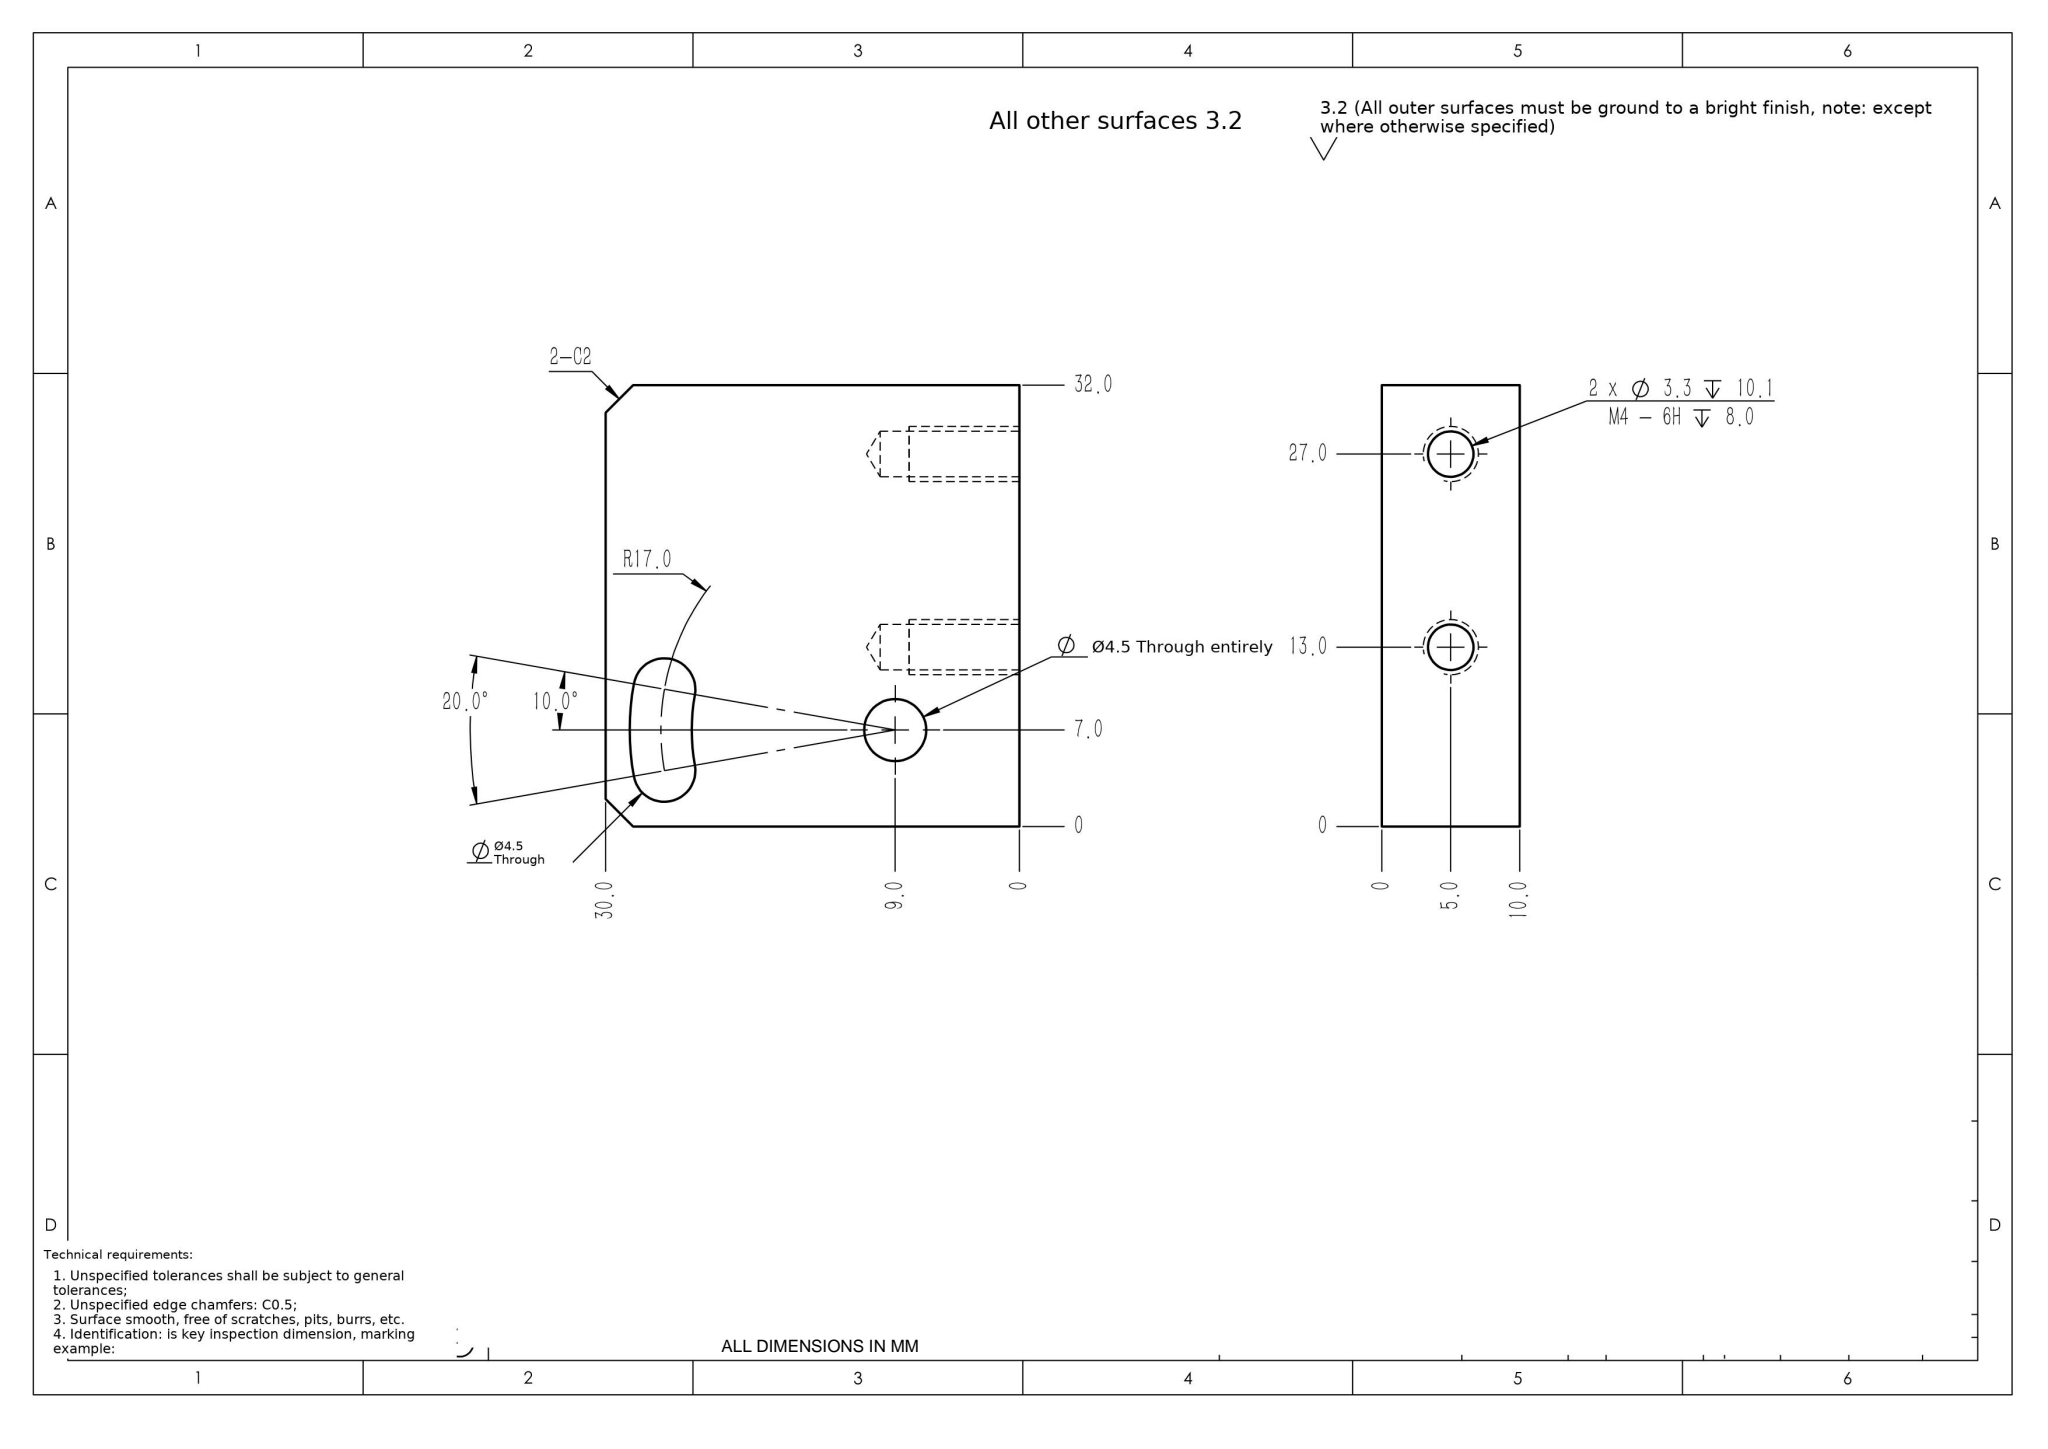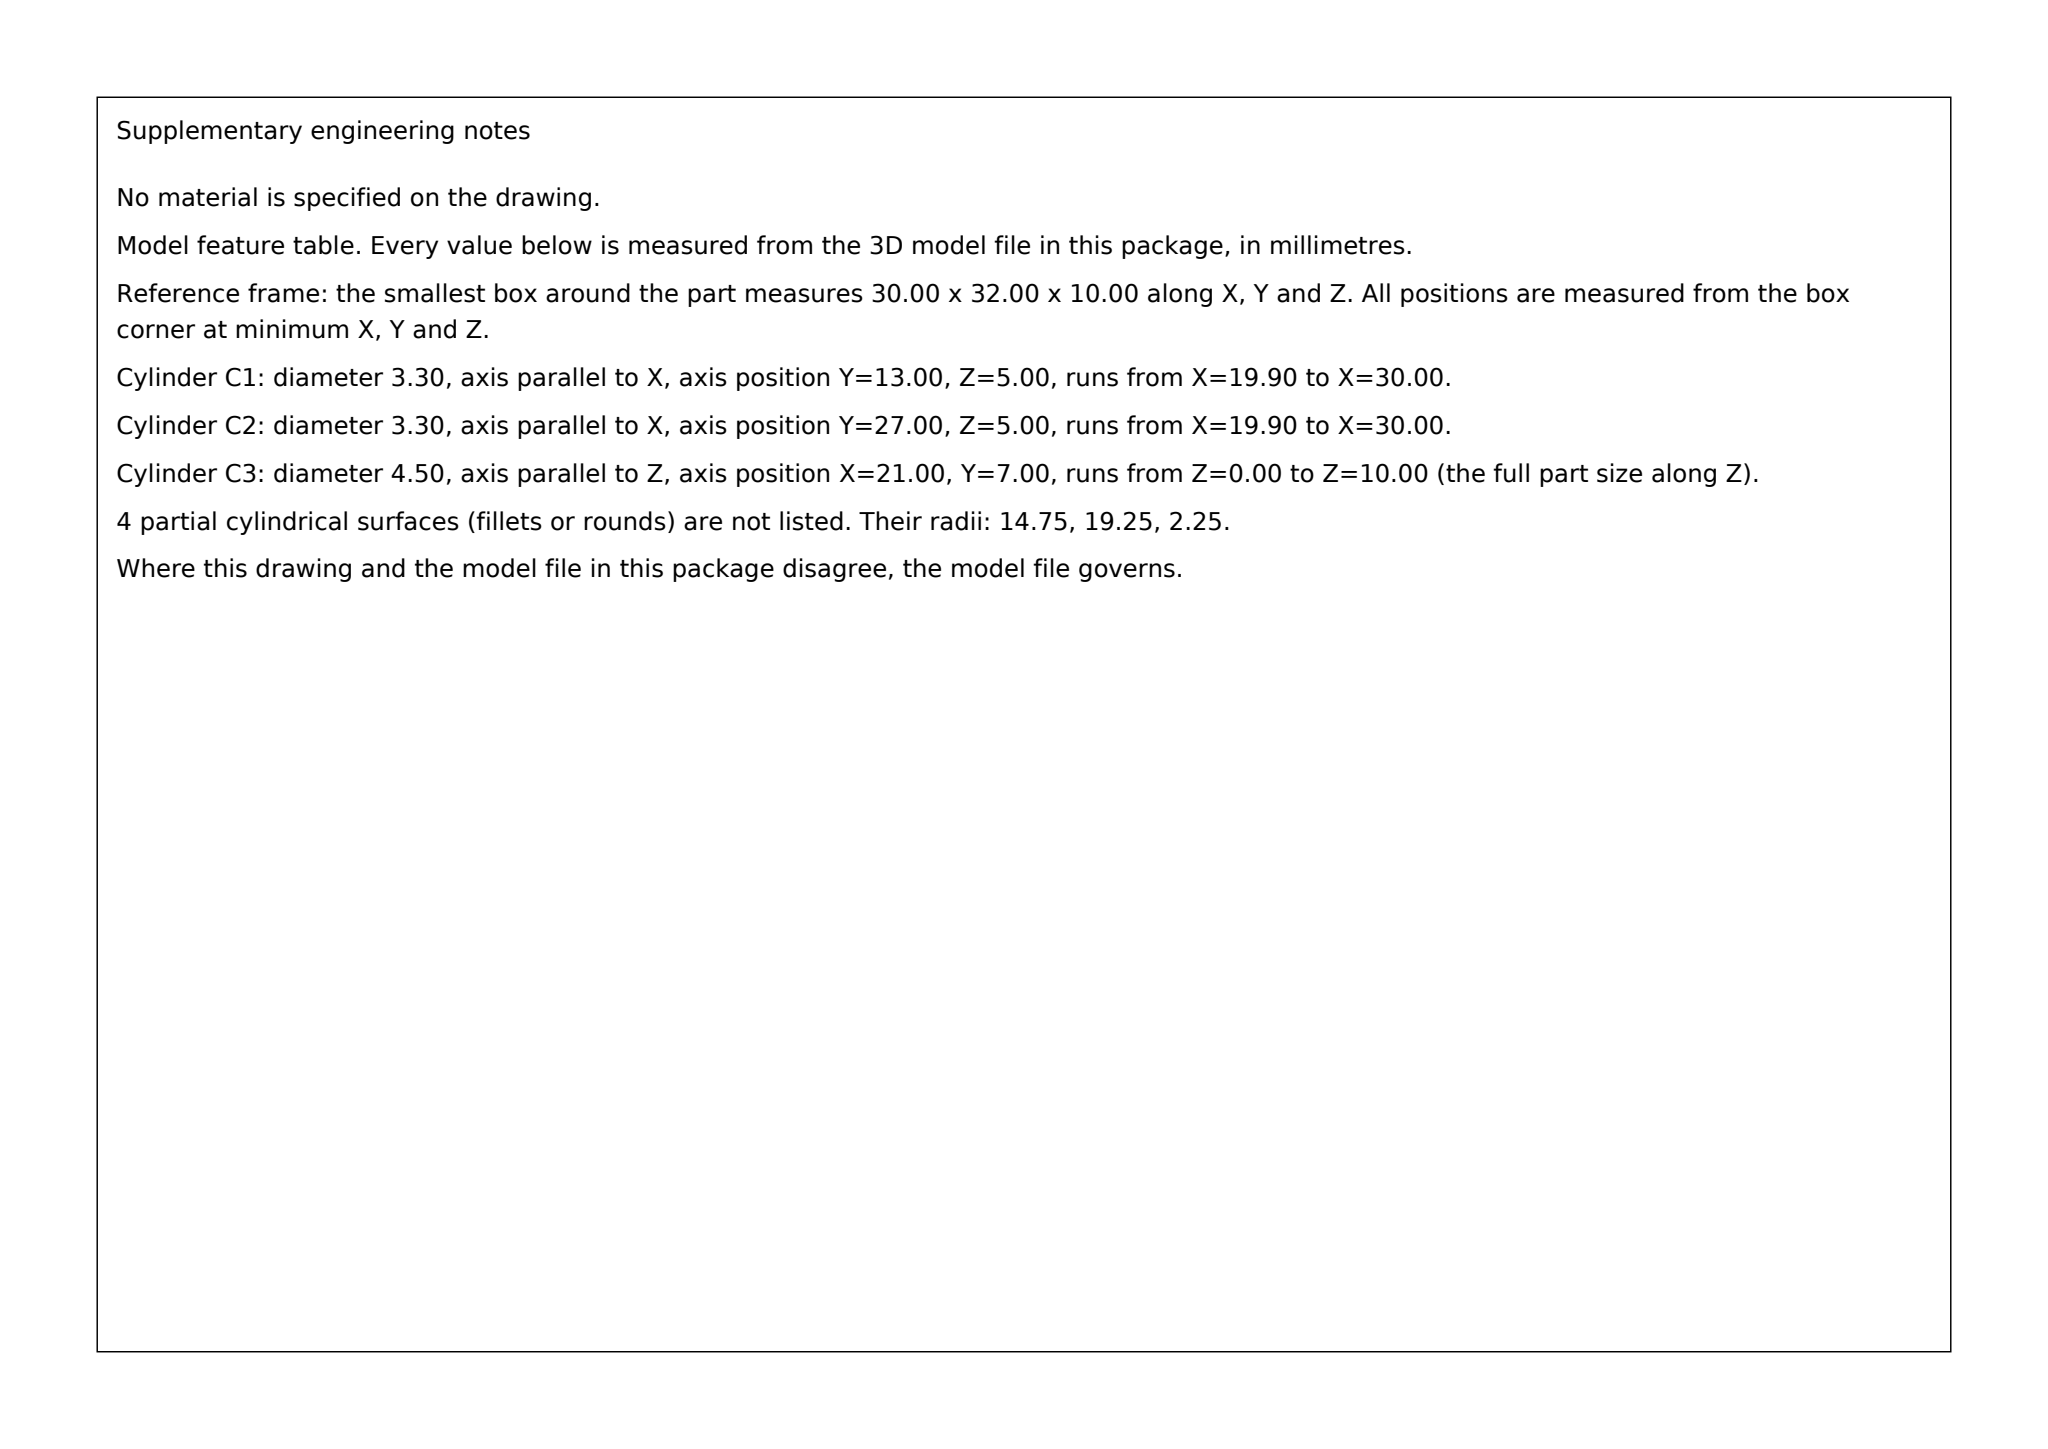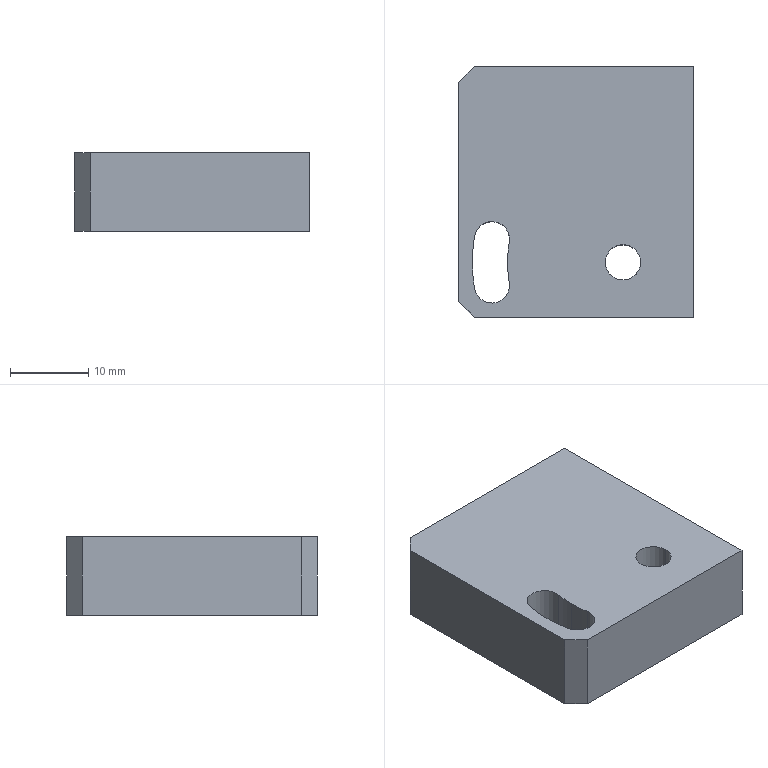Part | SolidWorks | mm | 1 solid | 24 faces | box 30 x 32 x 10 mm | volume 8796 mm3 | cylinder 12 | plane 8 | cone 4 | commonest cylinder face diameters 3.3 x4 4.5 x4 29.5 x2 38.5 x2
build123d program:
from build123d import *

# Parameters (mm, degrees)
SKETCH1_W             = 30
SKETCH1_H             = 32
BOSS_EXTRUDE1_DEPTH   = 10
M4_CLEARANCE_HOLE1_D  = 4.5
CUT_EXTRUDE3_DEPTH    = 25.104
CHAMFER1_SIZE         = 2
M4_TAPPED_HOLE2_D     = 3.3
M4_TAPPED_HOLE2_DEPTH = 10.1
M4_TAPPED_HOLE2_TIP   = 0.9914


with BuildPart() as part:
    # Sketch1 → Boss-Extrude1 (new body)
    with BuildSketch(Plane.XY):
        Rectangle(SKETCH1_W, SKETCH1_H)
    extrude(amount=BOSS_EXTRUDE1_DEPTH)

    # M4 Clearance Hole1 (through all)
    with Locations(Plane(origin=(0, 0, 0), x_dir=(-1, 0, 0), z_dir=(0, 0, -1))):
        with Locations((-6, -9)):
            Hole(M4_CLEARANCE_HOLE1_D / 2)

    # Sketch10 → Cut-Extrude3 (cut, through all)
    with BuildSketch(Plane(origin=(0, 0, 0), x_dir=(-1, 0, 0), z_dir=(0, 0, -1))):
        with BuildLine():
            ThreePointArc((12.958, -5.657), (10.351, -3.832), (8.526, -6.439))
            ThreePointArc((8.526, -6.439), (8.75, -9), (8.526, -11.561))
            ThreePointArc((8.526, -11.561), (10.351, -14.168), (12.958, -12.343))
            ThreePointArc((12.958, -12.343), (13.25, -9), (12.958, -5.657))
        make_face()
    extrude(amount=-CUT_EXTRUDE3_DEPTH, mode=Mode.SUBTRACT)

    # Chamfer1
    chamfer1_edges = [part.edges().sort_by_distance(p)[0] for p in [
        (-15, 16, 5),
        (-15, -16, 5),
    ]]
    chamfer(chamfer1_edges, length=CHAMFER1_SIZE)

    # M4 Tapped Hole2
    with Locations(Plane(origin=(15, 0, 0), x_dir=(0, 0, -1), z_dir=(1, 0, 0))):
        with Locations((-5, -3), (-5, 11)):
            Hole(M4_TAPPED_HOLE2_D / 2, depth=M4_TAPPED_HOLE2_DEPTH)
            with Locations((0, 0, -(M4_TAPPED_HOLE2_DEPTH + M4_TAPPED_HOLE2_TIP / 2))):  # 118° drill point
                Cone(0, M4_TAPPED_HOLE2_D / 2, M4_TAPPED_HOLE2_TIP, mode=Mode.SUBTRACT)


solid = part.part
STEP:
#1=CARTESIAN_POINT('',(4.9,-3.,6.65));
#2=VERTEX_POINT('',#1);
#3=CARTESIAN_POINT('',(4.9,-3.,3.35));
#4=VERTEX_POINT('',#3);
#5=CARTESIAN_POINT('',(4.9,-3.,5.));
#6=DIRECTION('',(1.,0.,0.));
#7=DIRECTION('',(0.,0.,-1.));
#8=AXIS2_PLACEMENT_3D('',#5,#6,#7);
#9=CIRCLE('',#8,1.65);
#10=EDGE_CURVE('',#2,#4,#9,.T.);
#11=ORIENTED_EDGE('',*,*,#10,.F.);
#12=CARTESIAN_POINT('',(15.,-3.,6.65));
#13=VERTEX_POINT('',#12);
#14=CARTESIAN_POINT('',(15.,-3.,6.65));
#15=DIRECTION('',(1.,0.,0.));
#16=VECTOR('',#15,1000.);
#17=LINE('',#14,#16);
#18=EDGE_CURVE('',#2,#13,#17,.T.);
#19=ORIENTED_EDGE('',*,*,#18,.T.);
#20=CARTESIAN_POINT('',(15.,-3.,3.35));
#21=VERTEX_POINT('',#20);
#22=CARTESIAN_POINT('',(15.,-3.,5.));
#23=DIRECTION('',(1.,0.,0.));
#24=DIRECTION('',(0.,0.,-1.));
#25=AXIS2_PLACEMENT_3D('',#22,#23,#24);
#26=CIRCLE('',#25,1.65);
#27=EDGE_CURVE('',#13,#21,#26,.T.);
#28=ORIENTED_EDGE('',*,*,#27,.T.);
#29=CARTESIAN_POINT('',(15.,-3.,3.35));
#30=DIRECTION('',(1.,0.,0.));
#31=VECTOR('',#30,1000.);
#32=LINE('',#29,#31);
#33=EDGE_CURVE('',#4,#21,#32,.T.);
#34=ORIENTED_EDGE('',*,*,#33,.F.);
#35=EDGE_LOOP('',(#11,#19,#28,#34));
#36=FACE_OUTER_BOUND('',#35,.T.);
#37=CARTESIAN_POINT('',(15.,-3.,5.));
#38=DIRECTION('',(1.,0.,0.));
#39=DIRECTION('',(0.,0.,-1.));
#40=AXIS2_PLACEMENT_3D('',#37,#38,#39);
#41=CYLINDRICAL_SURFACE('',#40,1.65);
#42=ADVANCED_FACE('',(#36),#41,.F.);
#43=CARTESIAN_POINT('',(3.909,-3.,5.));
#44=VERTEX_POINT('',#43);
#45=CARTESIAN_POINT('',(4.9,-3.,3.35));
#46=DIRECTION('',(0.515,0.,-0.8572));
#47=VECTOR('',#46,1000.);
#48=LINE('',#45,#47);
#49=EDGE_CURVE('',#44,#4,#48,.T.);
#50=ORIENTED_EDGE('',*,*,#49,.F.);
#51=CARTESIAN_POINT('',(4.9,-3.,6.65));
#52=DIRECTION('',(0.515,0.,0.8572));
#53=VECTOR('',#52,1000.);
#54=LINE('',#51,#53);
#55=EDGE_CURVE('',#44,#2,#54,.T.);
#56=ORIENTED_EDGE('',*,*,#55,.T.);
#57=ORIENTED_EDGE('',*,*,#10,.T.);
#58=EDGE_LOOP('',(#50,#56,#57));
#59=FACE_OUTER_BOUND('',#58,.T.);
#60=CARTESIAN_POINT('',(4.9,-3.,5.));
#61=DIRECTION('',(1.,0.,0.));
#62=DIRECTION('',(0.,0.,-1.));
#63=AXIS2_PLACEMENT_3D('',#60,#61,#62);
#64=CONICAL_SURFACE('',#63,1.65,1.03);
#65=ADVANCED_FACE('',(#59),#64,.F.);
#66=CARTESIAN_POINT('',(4.9,11.,6.65));
#67=VERTEX_POINT('',#66);
#68=CARTESIAN_POINT('',(4.9,11.,3.35));
#69=VERTEX_POINT('',#68);
#70=CARTESIAN_POINT('',(4.9,11.,5.));
#71=DIRECTION('',(1.,0.,0.));
#72=DIRECTION('',(0.,0.,-1.));
#73=AXIS2_PLACEMENT_3D('',#70,#71,#72);
#74=CIRCLE('',#73,1.65);
#75=EDGE_CURVE('',#67,#69,#74,.T.);
#76=ORIENTED_EDGE('',*,*,#75,.F.);
#77=CARTESIAN_POINT('',(15.,11.,6.65));
#78=VERTEX_POINT('',#77);
#79=CARTESIAN_POINT('',(15.,11.,6.65));
#80=DIRECTION('',(1.,0.,0.));
#81=VECTOR('',#80,1000.);
#82=LINE('',#79,#81);
#83=EDGE_CURVE('',#67,#78,#82,.T.);
#84=ORIENTED_EDGE('',*,*,#83,.T.);
#85=CARTESIAN_POINT('',(15.,11.,3.35));
#86=VERTEX_POINT('',#85);
#87=CARTESIAN_POINT('',(15.,11.,5.));
#88=DIRECTION('',(1.,0.,0.));
#89=DIRECTION('',(0.,0.,-1.));
#90=AXIS2_PLACEMENT_3D('',#87,#88,#89);
#91=CIRCLE('',#90,1.65);
#92=EDGE_CURVE('',#78,#86,#91,.T.);
#93=ORIENTED_EDGE('',*,*,#92,.T.);
#94=CARTESIAN_POINT('',(15.,11.,3.35));
#95=DIRECTION('',(1.,0.,0.));
#96=VECTOR('',#95,1000.);
#97=LINE('',#94,#96);
#98=EDGE_CURVE('',#69,#86,#97,.T.);
#99=ORIENTED_EDGE('',*,*,#98,.F.);
#100=EDGE_LOOP('',(#76,#84,#93,#99));
#101=FACE_OUTER_BOUND('',#100,.T.);
#102=CARTESIAN_POINT('',(15.,11.,5.));
#103=DIRECTION('',(1.,0.,0.));
#104=DIRECTION('',(0.,0.,-1.));
#105=AXIS2_PLACEMENT_3D('',#102,#103,#104);
#106=CYLINDRICAL_SURFACE('',#105,1.65);
#107=ADVANCED_FACE('',(#101),#106,.F.);
#108=CARTESIAN_POINT('',(3.909,11.,5.));
#109=VERTEX_POINT('',#108);
#110=CARTESIAN_POINT('',(4.9,11.,3.35));
#111=DIRECTION('',(0.515,0.,-0.8572));
#112=VECTOR('',#111,1000.);
#113=LINE('',#110,#112);
#114=EDGE_CURVE('',#109,#69,#113,.T.);
#115=ORIENTED_EDGE('',*,*,#114,.F.);
#116=CARTESIAN_POINT('',(4.9,11.,6.65));
#117=DIRECTION('',(0.515,0.,0.8572));
#118=VECTOR('',#117,1000.);
#119=LINE('',#116,#118);
#120=EDGE_CURVE('',#109,#67,#119,.T.);
#121=ORIENTED_EDGE('',*,*,#120,.T.);
#122=ORIENTED_EDGE('',*,*,#75,.T.);
#123=EDGE_LOOP('',(#115,#121,#122));
#124=FACE_OUTER_BOUND('',#123,.T.);
#125=CARTESIAN_POINT('',(4.9,11.,5.));
#126=DIRECTION('',(1.,0.,0.));
#127=DIRECTION('',(0.,0.,-1.));
#128=AXIS2_PLACEMENT_3D('',#125,#126,#127);
#129=CONICAL_SURFACE('',#128,1.65,1.03);
#130=ADVANCED_FACE('',(#124),#129,.F.);
#131=CARTESIAN_POINT('',(-8.75,-9.,10.));
#132=VERTEX_POINT('',#131);
#133=CARTESIAN_POINT('',(-8.526,-11.561,10.));
#134=VERTEX_POINT('',#133);
#135=CARTESIAN_POINT('',(6.,-9.,10.));
#136=DIRECTION('',(0.,0.,1.));
#137=DIRECTION('',(-1.,0.,0.));
#138=AXIS2_PLACEMENT_3D('',#135,#136,#137);
#139=CIRCLE('',#138,14.75);
#140=EDGE_CURVE('',#132,#134,#139,.T.);
#141=ORIENTED_EDGE('',*,*,#140,.F.);
#142=CARTESIAN_POINT('',(-8.75,-9.,0.));
#143=VERTEX_POINT('',#142);
#144=CARTESIAN_POINT('',(-8.75,-9.,10.));
#145=DIRECTION('',(0.,0.,-1.));
#146=VECTOR('',#145,1000.);
#147=LINE('',#144,#146);
#148=EDGE_CURVE('',#132,#143,#147,.T.);
#149=ORIENTED_EDGE('',*,*,#148,.T.);
#150=CARTESIAN_POINT('',(-8.526,-11.561,0.));
#151=VERTEX_POINT('',#150);
#152=CARTESIAN_POINT('',(6.,-9.,0.));
#153=DIRECTION('',(0.,0.,1.));
#154=DIRECTION('',(-1.,0.,0.));
#155=AXIS2_PLACEMENT_3D('',#152,#153,#154);
#156=CIRCLE('',#155,14.75);
#157=EDGE_CURVE('',#143,#151,#156,.T.);
#158=ORIENTED_EDGE('',*,*,#157,.T.);
#159=CARTESIAN_POINT('',(-8.526,-11.561,10.));
#160=DIRECTION('',(0.,0.,-1.));
#161=VECTOR('',#160,1000.);
#162=LINE('',#159,#161);
#163=EDGE_CURVE('',#134,#151,#162,.T.);
#164=ORIENTED_EDGE('',*,*,#163,.F.);
#165=EDGE_LOOP('',(#141,#149,#158,#164));
#166=FACE_OUTER_BOUND('',#165,.T.);
#167=CARTESIAN_POINT('',(6.,-9.,10.));
#168=DIRECTION('',(0.,0.,-1.));
#169=DIRECTION('',(-1.,0.,0.));
#170=AXIS2_PLACEMENT_3D('',#167,#168,#169);
#171=CYLINDRICAL_SURFACE('',#170,14.75);
#172=ADVANCED_FACE('',(#166),#171,.T.);
#173=CARTESIAN_POINT('',(-13.25,-9.,10.));
#174=VERTEX_POINT('',#173);
#175=CARTESIAN_POINT('',(-12.958,-5.657,10.));
#176=VERTEX_POINT('',#175);
#177=CARTESIAN_POINT('',(6.,-9.,10.));
#178=DIRECTION('',(0.,0.,-1.));
#179=DIRECTION('',(-1.,0.,0.));
#180=AXIS2_PLACEMENT_3D('',#177,#178,#179);
#181=CIRCLE('',#180,19.25);
#182=EDGE_CURVE('',#174,#176,#181,.T.);
#183=ORIENTED_EDGE('',*,*,#182,.F.);
#184=CARTESIAN_POINT('',(-13.25,-9.,0.));
#185=VERTEX_POINT('',#184);
#186=CARTESIAN_POINT('',(-13.25,-9.,10.));
#187=DIRECTION('',(0.,0.,-1.));
#188=VECTOR('',#187,1000.);
#189=LINE('',#186,#188);
#190=EDGE_CURVE('',#174,#185,#189,.T.);
#191=ORIENTED_EDGE('',*,*,#190,.T.);
#192=CARTESIAN_POINT('',(-12.958,-5.657,0.));
#193=VERTEX_POINT('',#192);
#194=CARTESIAN_POINT('',(6.,-9.,0.));
#195=DIRECTION('',(0.,0.,-1.));
#196=DIRECTION('',(-1.,0.,0.));
#197=AXIS2_PLACEMENT_3D('',#194,#195,#196);
#198=CIRCLE('',#197,19.25);
#199=EDGE_CURVE('',#185,#193,#198,.T.);
#200=ORIENTED_EDGE('',*,*,#199,.T.);
#201=CARTESIAN_POINT('',(-12.958,-5.657,10.));
#202=DIRECTION('',(0.,0.,-1.));
#203=VECTOR('',#202,1000.);
#204=LINE('',#201,#203);
#205=EDGE_CURVE('',#176,#193,#204,.T.);
#206=ORIENTED_EDGE('',*,*,#205,.F.);
#207=EDGE_LOOP('',(#183,#191,#200,#206));
#208=FACE_OUTER_BOUND('',#207,.T.);
#209=CARTESIAN_POINT('',(6.,-9.,10.));
#210=DIRECTION('',(0.,0.,-1.));
#211=DIRECTION('',(-1.,0.,0.));
#212=AXIS2_PLACEMENT_3D('',#209,#210,#211);
#213=CYLINDRICAL_SURFACE('',#212,19.25);
#214=ADVANCED_FACE('',(#208),#213,.F.);
#215=CARTESIAN_POINT('',(8.25,-9.,10.));
#216=VERTEX_POINT('',#215);
#217=CARTESIAN_POINT('',(3.75,-9.,10.));
#218=VERTEX_POINT('',#217);
#219=CARTESIAN_POINT('',(6.,-9.,10.));
#220=DIRECTION('',(0.,0.,-1.));
#221=DIRECTION('',(-1.,0.,0.));
#222=AXIS2_PLACEMENT_3D('',#219,#220,#221);
#223=CIRCLE('',#222,2.25);
#224=EDGE_CURVE('',#216,#218,#223,.T.);
#225=ORIENTED_EDGE('',*,*,#224,.F.);
#226=CARTESIAN_POINT('',(8.25,-9.,-0.));
#227=VERTEX_POINT('',#226);
#228=CARTESIAN_POINT('',(8.25,-9.,0.));
#229=DIRECTION('',(0.,0.,-1.));
#230=VECTOR('',#229,1000.);
#231=LINE('',#228,#230);
#232=EDGE_CURVE('',#216,#227,#231,.T.);
#233=ORIENTED_EDGE('',*,*,#232,.T.);
#234=CARTESIAN_POINT('',(3.75,-9.,-0.));
#235=VERTEX_POINT('',#234);
#236=CARTESIAN_POINT('',(6.,-9.,-0.));
#237=DIRECTION('',(0.,0.,-1.));
#238=DIRECTION('',(-1.,0.,0.));
#239=AXIS2_PLACEMENT_3D('',#236,#237,#238);
#240=CIRCLE('',#239,2.25);
#241=EDGE_CURVE('',#227,#235,#240,.T.);
#242=ORIENTED_EDGE('',*,*,#241,.T.);
#243=CARTESIAN_POINT('',(3.75,-9.,0.));
#244=DIRECTION('',(0.,0.,-1.));
#245=VECTOR('',#244,1000.);
#246=LINE('',#243,#245);
#247=EDGE_CURVE('',#218,#235,#246,.T.);
#248=ORIENTED_EDGE('',*,*,#247,.F.);
#249=EDGE_LOOP('',(#225,#233,#242,#248));
#250=FACE_OUTER_BOUND('',#249,.T.);
#251=CARTESIAN_POINT('',(6.,-9.,0.));
#252=DIRECTION('',(0.,0.,-1.));
#253=DIRECTION('',(-1.,0.,0.));
#254=AXIS2_PLACEMENT_3D('',#251,#252,#253);
#255=CYLINDRICAL_SURFACE('',#254,2.25);
#256=ADVANCED_FACE('',(#250),#255,.F.);
#257=CARTESIAN_POINT('',(-15.,14.,10.));
#258=VERTEX_POINT('',#257);
#259=CARTESIAN_POINT('',(-15.,-14.,10.));
#260=VERTEX_POINT('',#259);
#261=CARTESIAN_POINT('',(-15.,16.,10.));
#262=DIRECTION('',(0.,-1.,0.));
#263=VECTOR('',#262,1000.);
#264=LINE('',#261,#263);
#265=EDGE_CURVE('',#258,#260,#264,.T.);
#266=ORIENTED_EDGE('',*,*,#265,.F.);
#267=CARTESIAN_POINT('',(-15.,14.,0.));
#268=VERTEX_POINT('',#267);
#269=CARTESIAN_POINT('',(-15.,14.,10.));
#270=DIRECTION('',(0.,0.,-1.));
#271=VECTOR('',#270,1000.);
#272=LINE('',#269,#271);
#273=EDGE_CURVE('',#258,#268,#272,.T.);
#274=ORIENTED_EDGE('',*,*,#273,.T.);
#275=CARTESIAN_POINT('',(-15.,-14.,0.));
#276=VERTEX_POINT('',#275);
#277=CARTESIAN_POINT('',(-15.,16.,0.));
#278=DIRECTION('',(0.,-1.,0.));
#279=VECTOR('',#278,1000.);
#280=LINE('',#277,#279);
#281=EDGE_CURVE('',#268,#276,#280,.T.);
#282=ORIENTED_EDGE('',*,*,#281,.T.);
#283=CARTESIAN_POINT('',(-15.,-14.,10.));
#284=DIRECTION('',(0.,0.,1.));
#285=VECTOR('',#284,1000.);
#286=LINE('',#283,#285);
#287=EDGE_CURVE('',#276,#260,#286,.T.);
#288=ORIENTED_EDGE('',*,*,#287,.T.);
#289=EDGE_LOOP('',(#266,#274,#282,#288));
#290=FACE_OUTER_BOUND('',#289,.T.);
#291=CARTESIAN_POINT('',(-15.,16.,10.));
#292=DIRECTION('',(1.,0.,0.));
#293=DIRECTION('',(-0.,1.,0.));
#294=AXIS2_PLACEMENT_3D('',#291,#292,#293);
#295=PLANE('',#294);
#296=ADVANCED_FACE('',(#290),#295,.F.);
#297=CARTESIAN_POINT('',(-13.,-16.,10.));
#298=VERTEX_POINT('',#297);
#299=CARTESIAN_POINT('',(15.,-16.,10.));
#300=VERTEX_POINT('',#299);
#301=CARTESIAN_POINT('',(15.,-16.,10.));
#302=DIRECTION('',(1.,0.,0.));
#303=VECTOR('',#302,1000.);
#304=LINE('',#301,#303);
#305=EDGE_CURVE('',#298,#300,#304,.T.);
#306=ORIENTED_EDGE('',*,*,#305,.F.);
#307=CARTESIAN_POINT('',(-13.,-16.,0.));
#308=VERTEX_POINT('',#307);
#309=CARTESIAN_POINT('',(-13.,-16.,10.));
#310=DIRECTION('',(0.,0.,-1.));
#311=VECTOR('',#310,1000.);
#312=LINE('',#309,#311);
#313=EDGE_CURVE('',#298,#308,#312,.T.);
#314=ORIENTED_EDGE('',*,*,#313,.T.);
#315=CARTESIAN_POINT('',(15.,-16.,0.));
#316=VERTEX_POINT('',#315);
#317=CARTESIAN_POINT('',(15.,-16.,0.));
#318=DIRECTION('',(1.,0.,0.));
#319=VECTOR('',#318,1000.);
#320=LINE('',#317,#319);
#321=EDGE_CURVE('',#308,#316,#320,.T.);
#322=ORIENTED_EDGE('',*,*,#321,.T.);
#323=CARTESIAN_POINT('',(15.,-16.,10.));
#324=DIRECTION('',(0.,0.,-1.));
#325=VECTOR('',#324,1000.);
#326=LINE('',#323,#325);
#327=EDGE_CURVE('',#300,#316,#326,.T.);
#328=ORIENTED_EDGE('',*,*,#327,.F.);
#329=EDGE_LOOP('',(#306,#314,#322,#328));
#330=FACE_OUTER_BOUND('',#329,.T.);
#331=CARTESIAN_POINT('',(15.,-16.,10.));
#332=DIRECTION('',(-0.,1.,0.));
#333=DIRECTION('',(-1.,-0.,0.));
#334=AXIS2_PLACEMENT_3D('',#331,#332,#333);
#335=PLANE('',#334);
#336=ADVANCED_FACE('',(#330),#335,.F.);
#337=CARTESIAN_POINT('',(15.,-3.,5.));
#338=DIRECTION('',(1.,0.,0.));
#339=DIRECTION('',(0.,0.,-1.));
#340=AXIS2_PLACEMENT_3D('',#337,#338,#339);
#341=CIRCLE('',#340,1.65);
#342=EDGE_CURVE('',#21,#13,#341,.T.);
#343=ORIENTED_EDGE('',*,*,#342,.F.);
#344=ORIENTED_EDGE('',*,*,#27,.F.);
#345=EDGE_LOOP('',(#343,#344));
#346=FACE_BOUND('',#345,.T.);
#347=CARTESIAN_POINT('',(15.,11.,5.));
#348=DIRECTION('',(1.,0.,0.));
#349=DIRECTION('',(0.,0.,-1.));
#350=AXIS2_PLACEMENT_3D('',#347,#348,#349);
#351=CIRCLE('',#350,1.65);
#352=EDGE_CURVE('',#86,#78,#351,.T.);
#353=ORIENTED_EDGE('',*,*,#352,.F.);
#354=ORIENTED_EDGE('',*,*,#92,.F.);
#355=EDGE_LOOP('',(#353,#354));
#356=FACE_BOUND('',#355,.T.);
#357=CARTESIAN_POINT('',(15.,16.,0.));
#358=VERTEX_POINT('',#357);
#359=CARTESIAN_POINT('',(15.,16.,0.));
#360=DIRECTION('',(-0.,1.,0.));
#361=VECTOR('',#360,1000.);
#362=LINE('',#359,#361);
#363=EDGE_CURVE('',#316,#358,#362,.T.);
#364=ORIENTED_EDGE('',*,*,#363,.T.);
#365=CARTESIAN_POINT('',(15.,16.,10.));
#366=VERTEX_POINT('',#365);
#367=CARTESIAN_POINT('',(15.,16.,10.));
#368=DIRECTION('',(0.,0.,-1.));
#369=VECTOR('',#368,1000.);
#370=LINE('',#367,#369);
#371=EDGE_CURVE('',#366,#358,#370,.T.);
#372=ORIENTED_EDGE('',*,*,#371,.F.);
#373=CARTESIAN_POINT('',(15.,16.,10.));
#374=DIRECTION('',(-0.,1.,0.));
#375=VECTOR('',#374,1000.);
#376=LINE('',#373,#375);
#377=EDGE_CURVE('',#300,#366,#376,.T.);
#378=ORIENTED_EDGE('',*,*,#377,.F.);
#379=ORIENTED_EDGE('',*,*,#327,.T.);
#380=EDGE_LOOP('',(#364,#372,#378,#379));
#381=FACE_OUTER_BOUND('',#380,.T.);
#382=CARTESIAN_POINT('',(15.,16.,10.));
#383=DIRECTION('',(-1.,-0.,0.));
#384=DIRECTION('',(0.,-1.,0.));
#385=AXIS2_PLACEMENT_3D('',#382,#383,#384);
#386=PLANE('',#385);
#387=ADVANCED_FACE('',(#346,#356,#381),#386,.F.);
#388=CARTESIAN_POINT('',(-13.,16.,0.));
#389=VERTEX_POINT('',#388);
#390=CARTESIAN_POINT('',(15.,16.,0.));
#391=DIRECTION('',(-1.,-0.,0.));
#392=VECTOR('',#391,1000.);
#393=LINE('',#390,#392);
#394=EDGE_CURVE('',#358,#389,#393,.T.);
#395=ORIENTED_EDGE('',*,*,#394,.T.);
#396=CARTESIAN_POINT('',(-13.,16.,10.));
#397=VERTEX_POINT('',#396);
#398=CARTESIAN_POINT('',(-13.,16.,10.));
#399=DIRECTION('',(0.,0.,1.));
#400=VECTOR('',#399,1000.);
#401=LINE('',#398,#400);
#402=EDGE_CURVE('',#389,#397,#401,.T.);
#403=ORIENTED_EDGE('',*,*,#402,.T.);
#404=CARTESIAN_POINT('',(15.,16.,10.));
#405=DIRECTION('',(-1.,-0.,0.));
#406=VECTOR('',#405,1000.);
#407=LINE('',#404,#406);
#408=EDGE_CURVE('',#366,#397,#407,.T.);
#409=ORIENTED_EDGE('',*,*,#408,.F.);
#410=ORIENTED_EDGE('',*,*,#371,.T.);
#411=EDGE_LOOP('',(#395,#403,#409,#410));
#412=FACE_OUTER_BOUND('',#411,.T.);
#413=CARTESIAN_POINT('',(15.,16.,10.));
#414=DIRECTION('',(0.,-1.,0.));
#415=DIRECTION('',(1.,0.,0.));
#416=AXIS2_PLACEMENT_3D('',#413,#414,#415);
#417=PLANE('',#416);
#418=ADVANCED_FACE('',(#412),#417,.F.);
#419=CARTESIAN_POINT('',(-12.958,-12.343,10.));
#420=VERTEX_POINT('',#419);
#421=CARTESIAN_POINT('',(-10.742,-11.952,10.));
#422=DIRECTION('',(0.,0.,-1.));
#423=DIRECTION('',(-1.,0.,0.));
#424=AXIS2_PLACEMENT_3D('',#421,#422,#423);
#425=CIRCLE('',#424,2.25);
#426=EDGE_CURVE('',#134,#420,#425,.T.);
#427=ORIENTED_EDGE('',*,*,#426,.T.);
#428=CARTESIAN_POINT('',(6.,-9.,10.));
#429=DIRECTION('',(0.,0.,-1.));
#430=DIRECTION('',(-1.,0.,0.));
#431=AXIS2_PLACEMENT_3D('',#428,#429,#430);
#432=CIRCLE('',#431,19.25);
#433=EDGE_CURVE('',#420,#174,#432,.T.);
#434=ORIENTED_EDGE('',*,*,#433,.T.);
#435=ORIENTED_EDGE('',*,*,#182,.T.);
#436=CARTESIAN_POINT('',(-8.526,-6.439,10.));
#437=VERTEX_POINT('',#436);
#438=CARTESIAN_POINT('',(-10.742,-6.048,10.));
#439=DIRECTION('',(0.,0.,-1.));
#440=DIRECTION('',(-1.,0.,0.));
#441=AXIS2_PLACEMENT_3D('',#438,#439,#440);
#442=CIRCLE('',#441,2.25);
#443=EDGE_CURVE('',#176,#437,#442,.T.);
#444=ORIENTED_EDGE('',*,*,#443,.T.);
#445=CARTESIAN_POINT('',(6.,-9.,10.));
#446=DIRECTION('',(0.,0.,1.));
#447=DIRECTION('',(-1.,0.,0.));
#448=AXIS2_PLACEMENT_3D('',#445,#446,#447);
#449=CIRCLE('',#448,14.75);
#450=EDGE_CURVE('',#437,#132,#449,.T.);
#451=ORIENTED_EDGE('',*,*,#450,.T.);
#452=ORIENTED_EDGE('',*,*,#140,.T.);
#453=EDGE_LOOP('',(#427,#434,#435,#444,#451,#452));
#454=FACE_BOUND('',#453,.T.);
#455=CARTESIAN_POINT('',(6.,-9.,10.));
#456=DIRECTION('',(0.,0.,-1.));
#457=DIRECTION('',(-1.,0.,0.));
#458=AXIS2_PLACEMENT_3D('',#455,#456,#457);
#459=CIRCLE('',#458,2.25);
#460=EDGE_CURVE('',#218,#216,#459,.T.);
#461=ORIENTED_EDGE('',*,*,#460,.T.);
#462=ORIENTED_EDGE('',*,*,#224,.T.);
#463=EDGE_LOOP('',(#461,#462));
#464=FACE_BOUND('',#463,.T.);
#465=ORIENTED_EDGE('',*,*,#408,.T.);
#466=CARTESIAN_POINT('',(-15.,14.,10.));
#467=DIRECTION('',(-0.7071,-0.7071,0.));
#468=VECTOR('',#467,1000.);
#469=LINE('',#466,#468);
#470=EDGE_CURVE('',#397,#258,#469,.T.);
#471=ORIENTED_EDGE('',*,*,#470,.T.);
#472=ORIENTED_EDGE('',*,*,#265,.T.);
#473=CARTESIAN_POINT('',(-13.,-16.,10.));
#474=DIRECTION('',(0.7071,-0.7071,0.));
#475=VECTOR('',#474,1000.);
#476=LINE('',#473,#475);
#477=EDGE_CURVE('',#260,#298,#476,.T.);
#478=ORIENTED_EDGE('',*,*,#477,.T.);
#479=ORIENTED_EDGE('',*,*,#305,.T.);
#480=ORIENTED_EDGE('',*,*,#377,.T.);
#481=EDGE_LOOP('',(#465,#471,#472,#478,#479,#480));
#482=FACE_OUTER_BOUND('',#481,.T.);
#483=CARTESIAN_POINT('',(0.,0.,10.));
#484=DIRECTION('',(0.,0.,-1.));
#485=DIRECTION('',(-1.,0.,0.));
#486=AXIS2_PLACEMENT_3D('',#483,#484,#485);
#487=PLANE('',#486);
#488=ADVANCED_FACE('',(#454,#464,#482),#487,.F.);
#489=CARTESIAN_POINT('',(-12.958,-12.343,0.));
#490=VERTEX_POINT('',#489);
#491=CARTESIAN_POINT('',(6.,-9.,0.));
#492=DIRECTION('',(0.,0.,-1.));
#493=DIRECTION('',(-1.,0.,0.));
#494=AXIS2_PLACEMENT_3D('',#491,#492,#493);
#495=CIRCLE('',#494,19.25);
#496=EDGE_CURVE('',#490,#185,#495,.T.);
#497=ORIENTED_EDGE('',*,*,#496,.F.);
#498=CARTESIAN_POINT('',(-10.742,-11.952,0.));
#499=DIRECTION('',(0.,0.,-1.));
#500=DIRECTION('',(-1.,0.,0.));
#501=AXIS2_PLACEMENT_3D('',#498,#499,#500);
#502=CIRCLE('',#501,2.25);
#503=EDGE_CURVE('',#151,#490,#502,.T.);
#504=ORIENTED_EDGE('',*,*,#503,.F.);
#505=ORIENTED_EDGE('',*,*,#157,.F.);
#506=CARTESIAN_POINT('',(-8.526,-6.439,0.));
#507=VERTEX_POINT('',#506);
#508=CARTESIAN_POINT('',(6.,-9.,0.));
#509=DIRECTION('',(0.,0.,1.));
#510=DIRECTION('',(-1.,0.,0.));
#511=AXIS2_PLACEMENT_3D('',#508,#509,#510);
#512=CIRCLE('',#511,14.75);
#513=EDGE_CURVE('',#507,#143,#512,.T.);
#514=ORIENTED_EDGE('',*,*,#513,.F.);
#515=CARTESIAN_POINT('',(-10.742,-6.048,0.));
#516=DIRECTION('',(0.,0.,-1.));
#517=DIRECTION('',(-1.,0.,0.));
#518=AXIS2_PLACEMENT_3D('',#515,#516,#517);
#519=CIRCLE('',#518,2.25);
#520=EDGE_CURVE('',#193,#507,#519,.T.);
#521=ORIENTED_EDGE('',*,*,#520,.F.);
#522=ORIENTED_EDGE('',*,*,#199,.F.);
#523=EDGE_LOOP('',(#497,#504,#505,#514,#521,#522));
#524=FACE_BOUND('',#523,.T.);
#525=CARTESIAN_POINT('',(6.,-9.,-0.));
#526=DIRECTION('',(0.,0.,-1.));
#527=DIRECTION('',(-1.,0.,0.));
#528=AXIS2_PLACEMENT_3D('',#525,#526,#527);
#529=CIRCLE('',#528,2.25);
#530=EDGE_CURVE('',#235,#227,#529,.T.);
#531=ORIENTED_EDGE('',*,*,#530,.F.);
#532=ORIENTED_EDGE('',*,*,#241,.F.);
#533=EDGE_LOOP('',(#531,#532));
#534=FACE_BOUND('',#533,.T.);
#535=ORIENTED_EDGE('',*,*,#281,.F.);
#536=CARTESIAN_POINT('',(-14.5,14.5,0.));
#537=DIRECTION('',(0.7071,0.7071,0.));
#538=VECTOR('',#537,1000.);
#539=LINE('',#536,#538);
#540=EDGE_CURVE('',#268,#389,#539,.T.);
#541=ORIENTED_EDGE('',*,*,#540,.T.);
#542=ORIENTED_EDGE('',*,*,#394,.F.);
#543=ORIENTED_EDGE('',*,*,#363,.F.);
#544=ORIENTED_EDGE('',*,*,#321,.F.);
#545=CARTESIAN_POINT('',(-14.5,-14.5,0.));
#546=DIRECTION('',(-0.7071,0.7071,0.));
#547=VECTOR('',#546,1000.);
#548=LINE('',#545,#547);
#549=EDGE_CURVE('',#308,#276,#548,.T.);
#550=ORIENTED_EDGE('',*,*,#549,.T.);
#551=EDGE_LOOP('',(#535,#541,#542,#543,#544,#550));
#552=FACE_OUTER_BOUND('',#551,.T.);
#553=CARTESIAN_POINT('',(0.,0.,0.));
#554=DIRECTION('',(0.,0.,-1.));
#555=DIRECTION('',(-1.,0.,0.));
#556=AXIS2_PLACEMENT_3D('',#553,#554,#555);
#557=PLANE('',#556);
#558=ADVANCED_FACE('',(#524,#534,#552),#557,.T.);
#559=ORIENTED_EDGE('',*,*,#232,.F.);
#560=ORIENTED_EDGE('',*,*,#460,.F.);
#561=ORIENTED_EDGE('',*,*,#247,.T.);
#562=ORIENTED_EDGE('',*,*,#530,.T.);
#563=EDGE_LOOP('',(#559,#560,#561,#562));
#564=FACE_OUTER_BOUND('',#563,.T.);
#565=CARTESIAN_POINT('',(6.,-9.,0.));
#566=DIRECTION('',(0.,0.,-1.));
#567=DIRECTION('',(-1.,0.,0.));
#568=AXIS2_PLACEMENT_3D('',#565,#566,#567);
#569=CYLINDRICAL_SURFACE('',#568,2.25);
#570=ADVANCED_FACE('',(#564),#569,.F.);
#571=ORIENTED_EDGE('',*,*,#190,.F.);
#572=ORIENTED_EDGE('',*,*,#433,.F.);
#573=CARTESIAN_POINT('',(-12.958,-12.343,10.));
#574=DIRECTION('',(0.,0.,-1.));
#575=VECTOR('',#574,1000.);
#576=LINE('',#573,#575);
#577=EDGE_CURVE('',#420,#490,#576,.T.);
#578=ORIENTED_EDGE('',*,*,#577,.T.);
#579=ORIENTED_EDGE('',*,*,#496,.T.);
#580=EDGE_LOOP('',(#571,#572,#578,#579));
#581=FACE_OUTER_BOUND('',#580,.T.);
#582=CARTESIAN_POINT('',(6.,-9.,10.));
#583=DIRECTION('',(0.,0.,-1.));
#584=DIRECTION('',(-1.,0.,0.));
#585=AXIS2_PLACEMENT_3D('',#582,#583,#584);
#586=CYLINDRICAL_SURFACE('',#585,19.25);
#587=ADVANCED_FACE('',(#581),#586,.F.);
#588=ORIENTED_EDGE('',*,*,#503,.T.);
#589=ORIENTED_EDGE('',*,*,#577,.F.);
#590=ORIENTED_EDGE('',*,*,#426,.F.);
#591=ORIENTED_EDGE('',*,*,#163,.T.);
#592=EDGE_LOOP('',(#588,#589,#590,#591));
#593=FACE_OUTER_BOUND('',#592,.T.);
#594=CARTESIAN_POINT('',(-10.742,-11.952,10.));
#595=DIRECTION('',(0.,0.,-1.));
#596=DIRECTION('',(-1.,0.,0.));
#597=AXIS2_PLACEMENT_3D('',#594,#595,#596);
#598=CYLINDRICAL_SURFACE('',#597,2.25);
#599=ADVANCED_FACE('',(#593),#598,.F.);
#600=ORIENTED_EDGE('',*,*,#148,.F.);
#601=ORIENTED_EDGE('',*,*,#450,.F.);
#602=CARTESIAN_POINT('',(-8.526,-6.439,10.));
#603=DIRECTION('',(0.,0.,-1.));
#604=VECTOR('',#603,1000.);
#605=LINE('',#602,#604);
#606=EDGE_CURVE('',#437,#507,#605,.T.);
#607=ORIENTED_EDGE('',*,*,#606,.T.);
#608=ORIENTED_EDGE('',*,*,#513,.T.);
#609=EDGE_LOOP('',(#600,#601,#607,#608));
#610=FACE_OUTER_BOUND('',#609,.T.);
#611=CARTESIAN_POINT('',(6.,-9.,10.));
#612=DIRECTION('',(0.,0.,-1.));
#613=DIRECTION('',(-1.,0.,0.));
#614=AXIS2_PLACEMENT_3D('',#611,#612,#613);
#615=CYLINDRICAL_SURFACE('',#614,14.75);
#616=ADVANCED_FACE('',(#610),#615,.T.);
#617=ORIENTED_EDGE('',*,*,#520,.T.);
#618=ORIENTED_EDGE('',*,*,#606,.F.);
#619=ORIENTED_EDGE('',*,*,#443,.F.);
#620=ORIENTED_EDGE('',*,*,#205,.T.);
#621=EDGE_LOOP('',(#617,#618,#619,#620));
#622=FACE_OUTER_BOUND('',#621,.T.);
#623=CARTESIAN_POINT('',(-10.742,-6.048,10.));
#624=DIRECTION('',(0.,0.,-1.));
#625=DIRECTION('',(-1.,0.,0.));
#626=AXIS2_PLACEMENT_3D('',#623,#624,#625);
#627=CYLINDRICAL_SURFACE('',#626,2.25);
#628=ADVANCED_FACE('',(#622),#627,.F.);
#629=ORIENTED_EDGE('',*,*,#470,.F.);
#630=ORIENTED_EDGE('',*,*,#402,.F.);
#631=ORIENTED_EDGE('',*,*,#540,.F.);
#632=ORIENTED_EDGE('',*,*,#273,.F.);
#633=EDGE_LOOP('',(#629,#630,#631,#632));
#634=FACE_OUTER_BOUND('',#633,.T.);
#635=CARTESIAN_POINT('',(-15.,14.,10.));
#636=DIRECTION('',(0.7071,-0.7071,0.));
#637=DIRECTION('',(0.,0.,-1.));
#638=AXIS2_PLACEMENT_3D('',#635,#636,#637);
#639=PLANE('',#638);
#640=ADVANCED_FACE('',(#634),#639,.F.);
#641=ORIENTED_EDGE('',*,*,#477,.F.);
#642=ORIENTED_EDGE('',*,*,#287,.F.);
#643=ORIENTED_EDGE('',*,*,#549,.F.);
#644=ORIENTED_EDGE('',*,*,#313,.F.);
#645=EDGE_LOOP('',(#641,#642,#643,#644));
#646=FACE_OUTER_BOUND('',#645,.T.);
#647=CARTESIAN_POINT('',(-13.,-16.,10.));
#648=DIRECTION('',(0.7071,0.7071,0.));
#649=DIRECTION('',(0.,0.,-1.));
#650=AXIS2_PLACEMENT_3D('',#647,#648,#649);
#651=PLANE('',#650);
#652=ADVANCED_FACE('',(#646),#651,.F.);
#653=ORIENTED_EDGE('',*,*,#120,.F.);
#654=ORIENTED_EDGE('',*,*,#114,.T.);
#655=CARTESIAN_POINT('',(4.9,11.,5.));
#656=DIRECTION('',(1.,0.,0.));
#657=DIRECTION('',(0.,0.,-1.));
#658=AXIS2_PLACEMENT_3D('',#655,#656,#657);
#659=CIRCLE('',#658,1.65);
#660=EDGE_CURVE('',#69,#67,#659,.T.);
#661=ORIENTED_EDGE('',*,*,#660,.T.);
#662=EDGE_LOOP('',(#653,#654,#661));
#663=FACE_OUTER_BOUND('',#662,.T.);
#664=CARTESIAN_POINT('',(4.9,11.,5.));
#665=DIRECTION('',(1.,0.,0.));
#666=DIRECTION('',(0.,0.,-1.));
#667=AXIS2_PLACEMENT_3D('',#664,#665,#666);
#668=CONICAL_SURFACE('',#667,1.65,1.03);
#669=ADVANCED_FACE('',(#663),#668,.F.);
#670=ORIENTED_EDGE('',*,*,#83,.F.);
#671=ORIENTED_EDGE('',*,*,#660,.F.);
#672=ORIENTED_EDGE('',*,*,#98,.T.);
#673=ORIENTED_EDGE('',*,*,#352,.T.);
#674=EDGE_LOOP('',(#670,#671,#672,#673));
#675=FACE_OUTER_BOUND('',#674,.T.);
#676=CARTESIAN_POINT('',(15.,11.,5.));
#677=DIRECTION('',(1.,0.,0.));
#678=DIRECTION('',(0.,0.,-1.));
#679=AXIS2_PLACEMENT_3D('',#676,#677,#678);
#680=CYLINDRICAL_SURFACE('',#679,1.65);
#681=ADVANCED_FACE('',(#675),#680,.F.);
#682=ORIENTED_EDGE('',*,*,#55,.F.);
#683=ORIENTED_EDGE('',*,*,#49,.T.);
#684=CARTESIAN_POINT('',(4.9,-3.,5.));
#685=DIRECTION('',(1.,0.,0.));
#686=DIRECTION('',(0.,0.,-1.));
#687=AXIS2_PLACEMENT_3D('',#684,#685,#686);
#688=CIRCLE('',#687,1.65);
#689=EDGE_CURVE('',#4,#2,#688,.T.);
#690=ORIENTED_EDGE('',*,*,#689,.T.);
#691=EDGE_LOOP('',(#682,#683,#690));
#692=FACE_OUTER_BOUND('',#691,.T.);
#693=CARTESIAN_POINT('',(4.9,-3.,5.));
#694=DIRECTION('',(1.,0.,0.));
#695=DIRECTION('',(0.,0.,-1.));
#696=AXIS2_PLACEMENT_3D('',#693,#694,#695);
#697=CONICAL_SURFACE('',#696,1.65,1.03);
#698=ADVANCED_FACE('',(#692),#697,.F.);
#699=ORIENTED_EDGE('',*,*,#18,.F.);
#700=ORIENTED_EDGE('',*,*,#689,.F.);
#701=ORIENTED_EDGE('',*,*,#33,.T.);
#702=ORIENTED_EDGE('',*,*,#342,.T.);
#703=EDGE_LOOP('',(#699,#700,#701,#702));
#704=FACE_OUTER_BOUND('',#703,.T.);
#705=CARTESIAN_POINT('',(15.,-3.,5.));
#706=DIRECTION('',(1.,0.,0.));
#707=DIRECTION('',(0.,0.,-1.));
#708=AXIS2_PLACEMENT_3D('',#705,#706,#707);
#709=CYLINDRICAL_SURFACE('',#708,1.65);
#710=ADVANCED_FACE('',(#704),#709,.F.);
#711=CLOSED_SHELL('',(#42,#65,#107,#130,#172,#214,#256,#296,#336,#387,#418,#488,#558,#570,#587,#599,#616,#628,#640,#652,#669,#681,#698,#710));
#712=MANIFOLD_SOLID_BREP('',#711);
#713=CARTESIAN_POINT('',(0.,0.,0.));
#714=DIRECTION('',(0.,0.,1.));
#715=DIRECTION('',(1.,0.,0.));
#716=AXIS2_PLACEMENT_3D('',#713,#714,#715);
#717=(LENGTH_UNIT()NAMED_UNIT(*)SI_UNIT(.MILLI.,.METRE.));
#718=UNCERTAINTY_MEASURE_WITH_UNIT(LENGTH_MEASURE(0.00001),#717,'','');
#719=(NAMED_UNIT(*)PLANE_ANGLE_UNIT()SI_UNIT($,.RADIAN.));
#720=(NAMED_UNIT(*)SI_UNIT($,.STERADIAN.)SOLID_ANGLE_UNIT());
#721=(GEOMETRIC_REPRESENTATION_CONTEXT(3)GLOBAL_UNCERTAINTY_ASSIGNED_CONTEXT((#718))GLOBAL_UNIT_ASSIGNED_CONTEXT((#717,#719,#720))REPRESENTATION_CONTEXT('',''));
#722=ADVANCED_BREP_SHAPE_REPRESENTATION('',(#712,#716),#721);